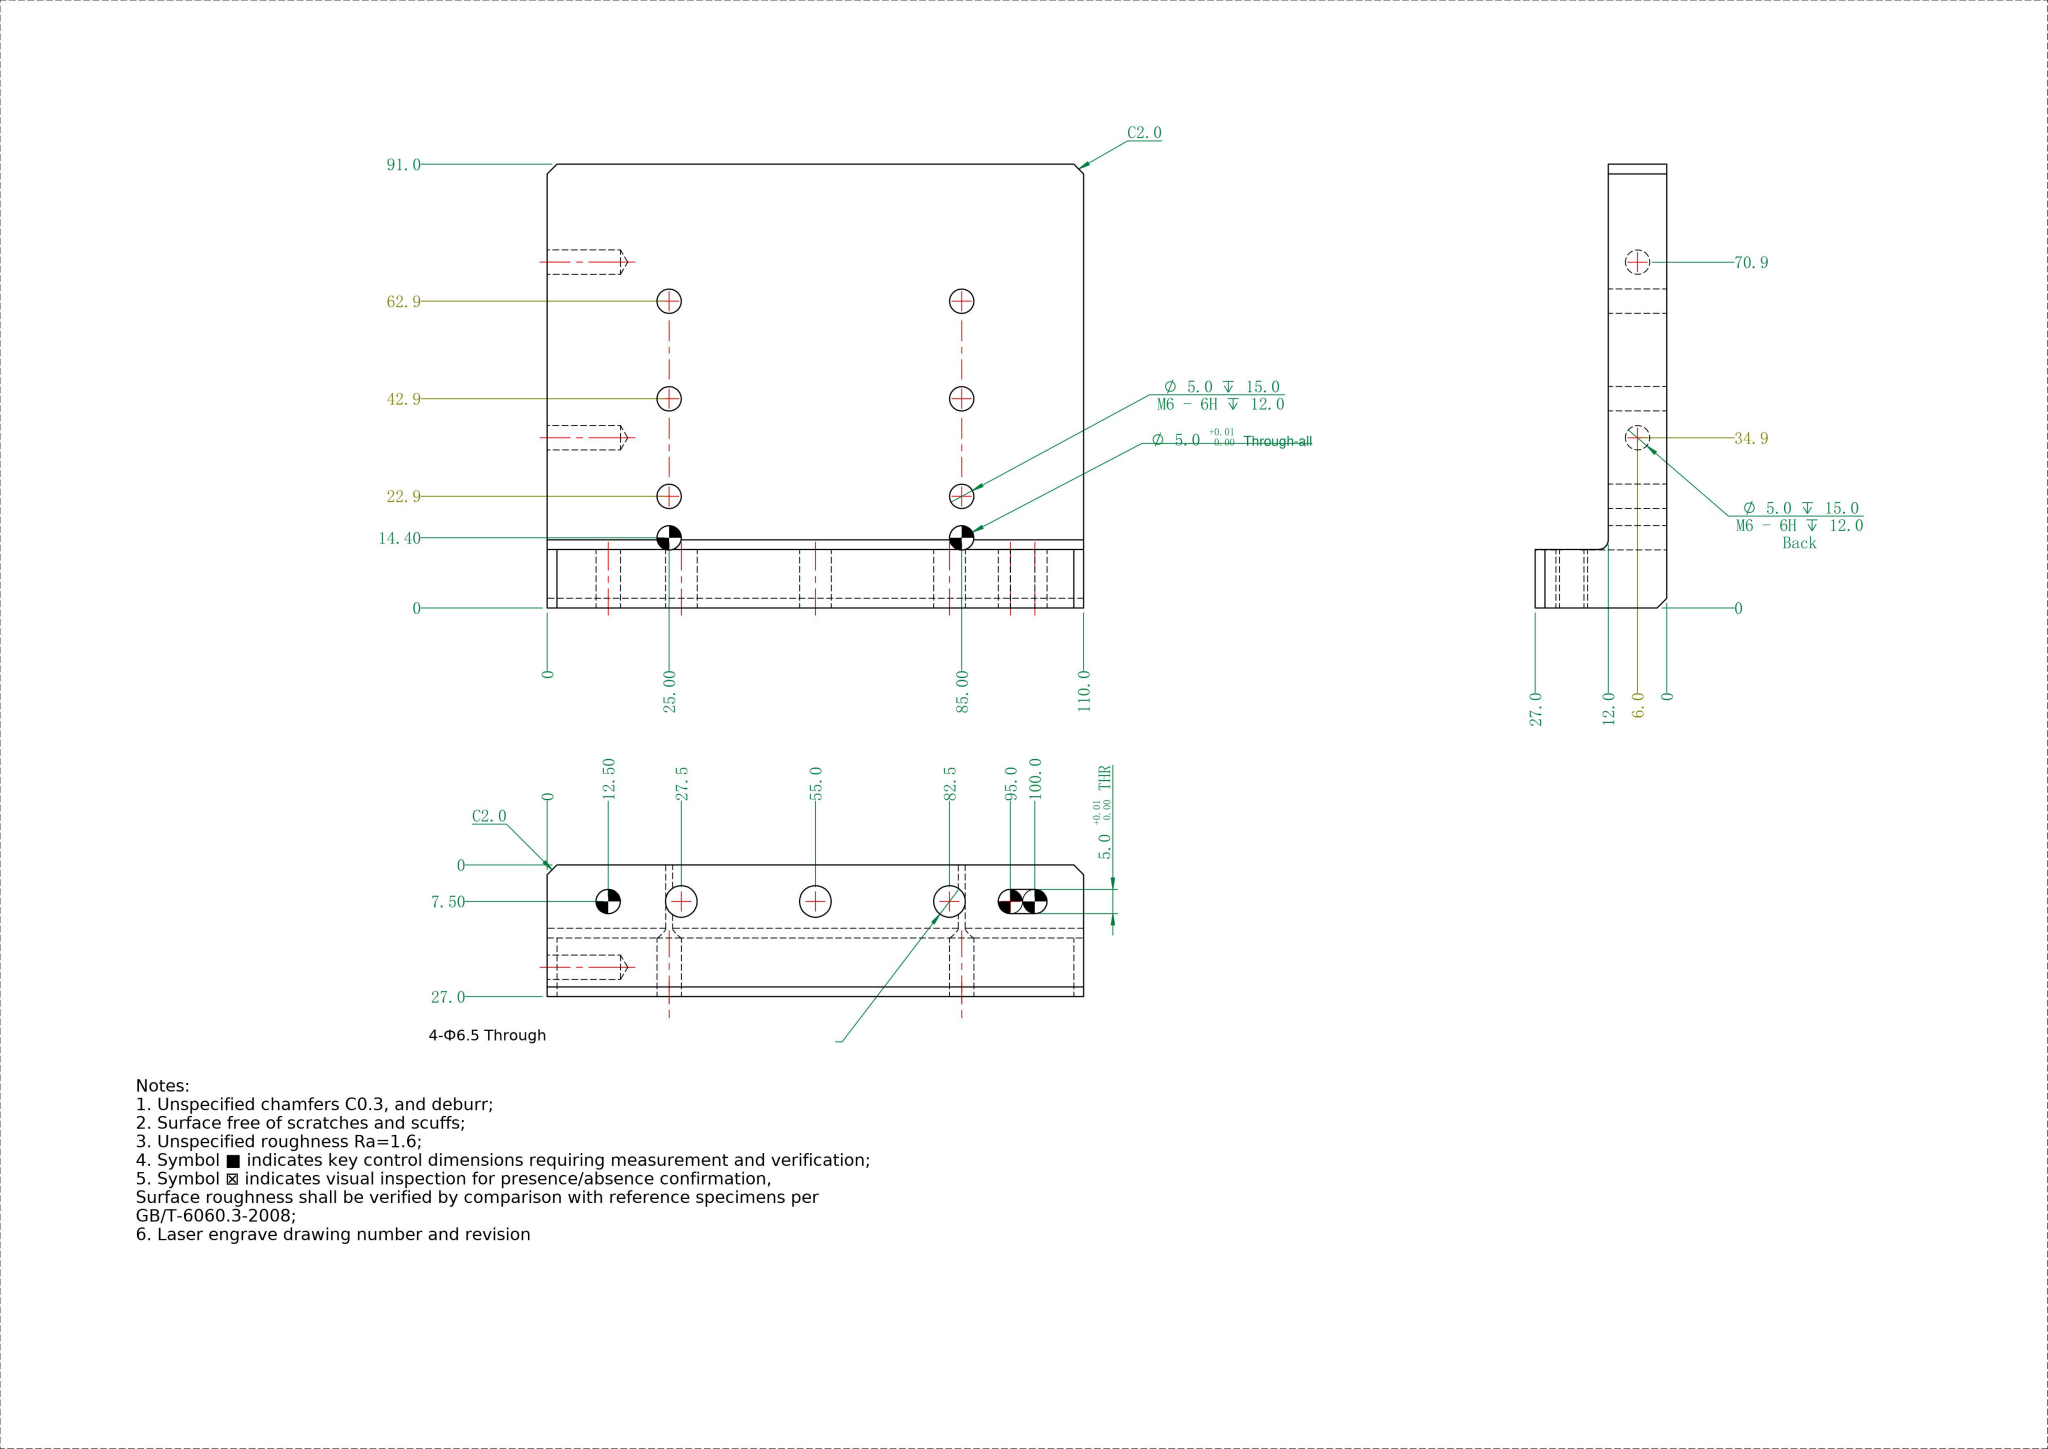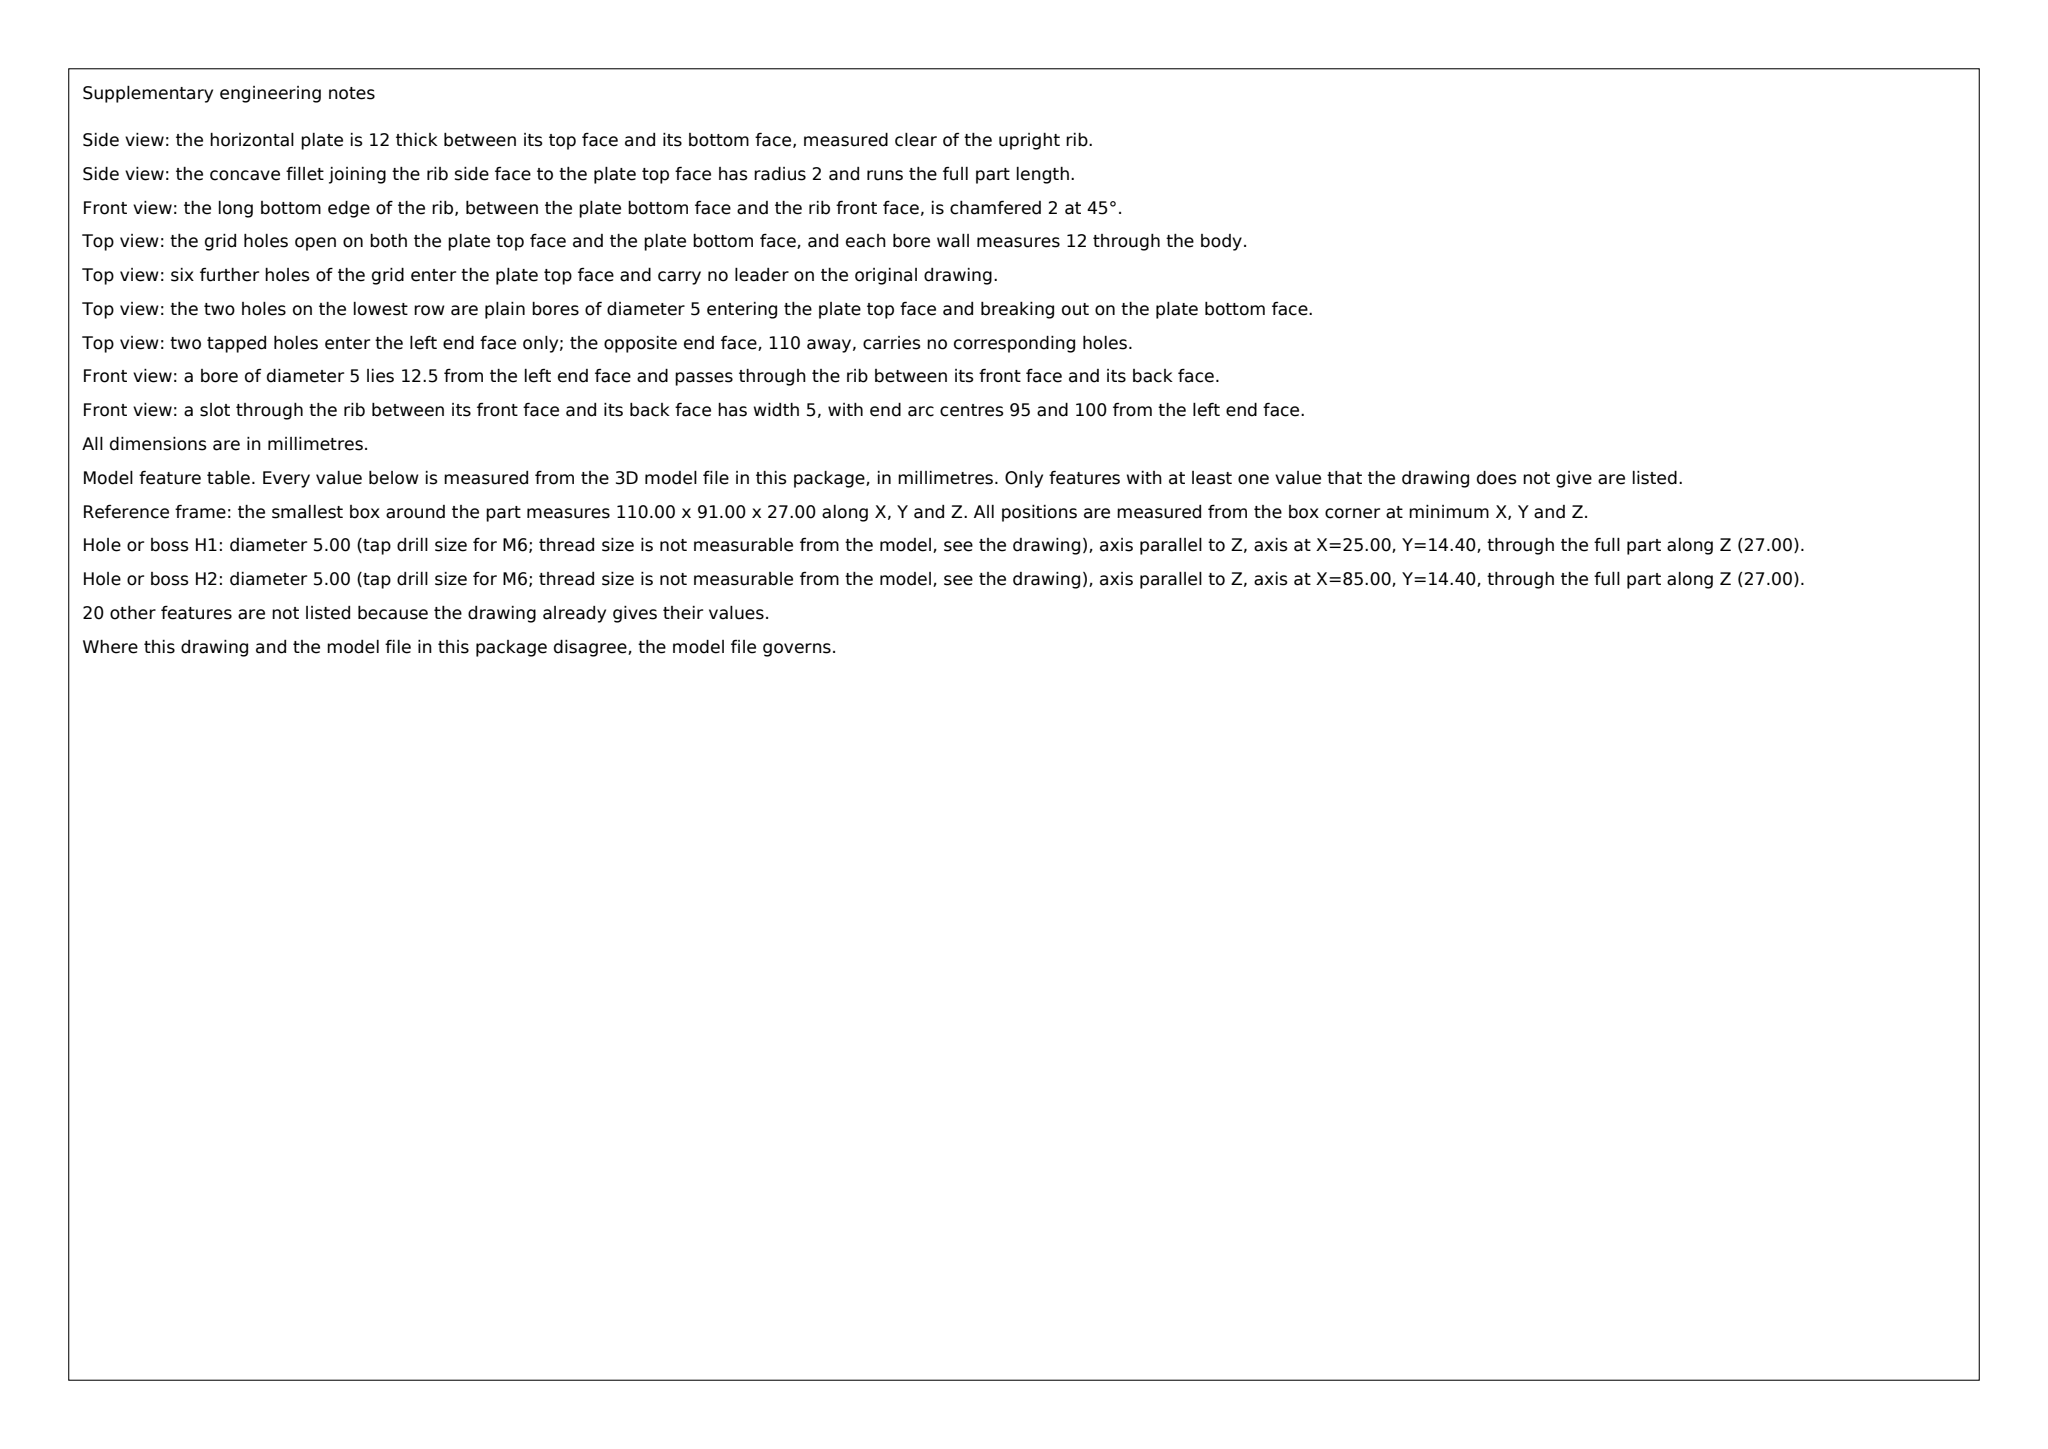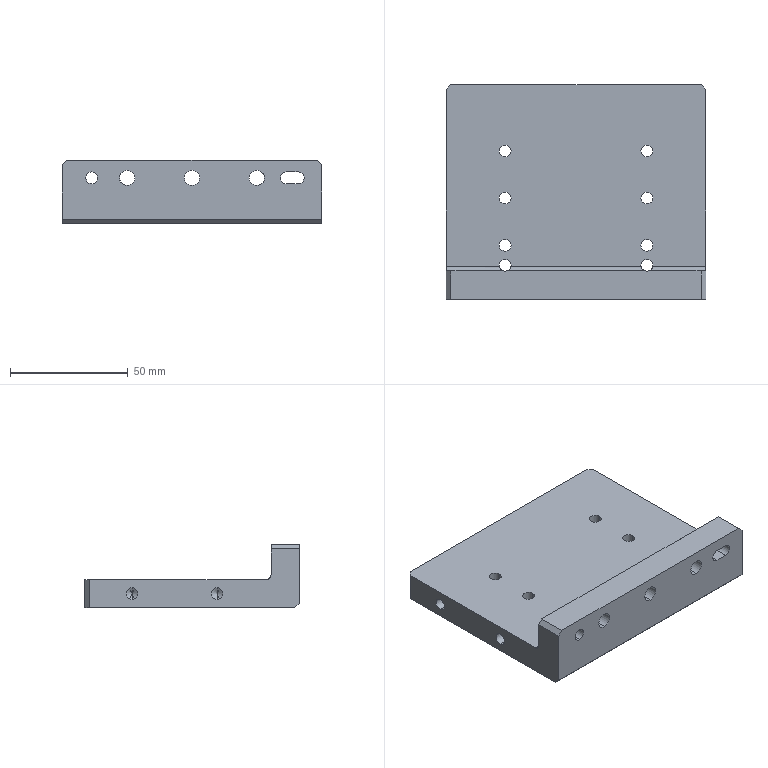Part | SolidWorks | mm | 1 solid | 56 faces | box 110 x 91 x 27 mm | volume 135232 mm3 | cylinder 35 | plane 17 | cone 4 | commonest cylinder face diameters 5 x26 6.5 x6 4 x3
Drawing notes:
3X Ø4.0 cross-hole, axis parallel to X at Y=14.0, Z=14.0 from the bbox min corner; segments X 0.0-24.3, X 25.7-84.3, X 85.7-110.0. | from the solid: cylinders: dia 4.0, axis x, axis_pos [-,14.0,14.0], from/to 0.0-24.3, 25.7-84.3, 85.7-110.0
Slot 5.0 wide THRU in Y (Y 0.0 to 12.0), flanks at Z=17.0 and Z=22.0, end radii centres at X=95.0 and X=100.0, Z=19.5 (7.5 below top face Z=27.0). | from the solid: axis_planes z=17.0 and z=22.0, extent x[95.0,100.0] y[0.0,12.0]; cylinders dia 5.0 axis y at [100.0,-,19.5] and [95.0,-,19.5], from 0.0 to 12.0
3X Ø6.5 THRU (not 4X), axis parallel to Y, Z=19.5, at X=27.5, 55.0 and 82.5; through Y 0.0 to 12.0. | from the solid: cylinders: dia 6.5, axis y, axis_pos [27.5/55.0/82.5, -, 19.5], from 0.0 to 12.0
All dimensions in millimetres (mm); overall size 110.0 x 91.0 x 27.0. | from the solid: bbox_xyz [110.0, 91.0, 27.0] (mm)
1X Ø5.0 THRU, axis parallel to Y, at X=12.5, Z=19.5 from bbox min corner; through Y 0.0 to 12.0 (12.0 deep). | from the solid: cylinders: hole/bore, dia 5.0, axis y, axis_pos [12.5, null, 19.5], from 0.0 to 12.0, arc 360
build123d program:
from build123d import *

# Parameters (mm, degrees)
SKETCH1_W                        = 110
SKETCH1_H                        = 91
BOSS_EXTRUDE1_DEPTH              = 12
SKETCH2_W                        = 110
SKETCH2_H                        = 12
BOSS_EXTRUDE2_DEPTH              = 15
FILLET1_R                        = 2
M6_TAPPED_HOLE1_D                = 5
M6_TAPPED_HOLE1_DEPTH            = 15
M6_TAPPED_HOLE1_TIP              = 1.502
M6_TAPPED_HOLE2_AT_2_COUNT       = 2
M6_TAPPED_HOLE2_AT_2_PITCH       = 60
LPATTERN1_COUNT                  = 3
LPATTERN1_PITCH                  = 20
CHAMFER1_SIZE                    = 2
CHAMFER2_SIZE                    = 2
SIZE_MM_DOWEL_PIN_HOLE_2_D       = 5
SKETCH9_R                        = 3.25
CUT_EXTRUDE1_DEPTH               = 100.975
SIZE_MM_DOWEL_PIN_HOLE_2_2_D     = 5
SIZE_MM_DOWEL_PIN_HOLE_2_2_DEPTH = 15
SIZE_MM_DOWEL_PIN_HOLE_2_2_TIP   = 1.502
CUT_EXTRUDE2_DEPTH               = 100.975


with BuildPart() as part:
    # Sketch1 → Boss-Extrude1 (new body)
    with BuildSketch(Plane.XY):
        Rectangle(SKETCH1_W, SKETCH1_H)
    extrude(amount=BOSS_EXTRUDE1_DEPTH)

    # Sketch2 → Boss-Extrude2 (add)
    with BuildSketch(Plane.XY.offset(12)):
        with Locations((0, -39.5)):
            Rectangle(SKETCH2_W, SKETCH2_H)
    extrude(amount=BOSS_EXTRUDE2_DEPTH)

    # Fillet1
    fillet1_edges = [part.edges().sort_by_distance(p)[0] for p in [
        (0, -33.5, 12),
    ]]
    fillet(fillet1_edges, radius=FILLET1_R)

    # M6 Tapped Hole1
    with Locations(Plane.ZY.offset(55)):
        with Locations((6, -10.6), (6, 25.4)):
            Hole(M6_TAPPED_HOLE1_D / 2, depth=M6_TAPPED_HOLE1_DEPTH)
            with Locations((0, 0, -(M6_TAPPED_HOLE1_DEPTH + M6_TAPPED_HOLE1_TIP / 2))):  # 118° drill point
                Cone(0, M6_TAPPED_HOLE1_D / 2, M6_TAPPED_HOLE1_TIP, mode=Mode.SUBTRACT)

    # Sketch6 → M6 Tapped Hole2 (revolve, cut)
    with BuildSketch(Plane(origin=(30, -22.6, 0), x_dir=(0, 1, 0), z_dir=(1, 0, 0))):
        Polygon((0, 0), (0, 16.502), (2.5, 15), (2.5, 0), align=None)
    m6_tapped_hole2 = revolve(axis=Axis((30, -22.6, -6.35), (0, 0, 1)), mode=Mode.SUBTRACT)

    # M6 Tapped Hole2 at 2: M6 Tapped Hole2 ×2
    with Locations(*[(-i * M6_TAPPED_HOLE2_AT_2_PITCH, 0, 0) for i in range(1, M6_TAPPED_HOLE2_AT_2_COUNT)]):
        add(m6_tapped_hole2, mode=Mode.SUBTRACT)

    # LPattern1: M6 Tapped Hole2 ×3
    with Locations(*[(0, i * LPATTERN1_PITCH, 0) for i in range(1, LPATTERN1_COUNT)]):
        add(m6_tapped_hole2, mode=Mode.SUBTRACT)

    # LPattern1 copy 1 sketch → LPattern1 copy 1 (revolve, cut)
    with BuildSketch(Plane(origin=(-30, -2.6, 0), x_dir=(0, 1, 0), z_dir=(1, 0, 0))):
        Polygon((0, 0), (0, 16.502), (2.5, 15), (2.5, 0), align=None)
    revolve(axis=Axis((-30, -2.6, -6.35), (0, 0, 1)), mode=Mode.SUBTRACT)

    # LPattern1 copy 2 sketch → LPattern1 copy 2 (revolve, cut)
    with BuildSketch(Plane(origin=(-30, 17.4, 0), x_dir=(0, 1, 0), z_dir=(1, 0, 0))):
        Polygon((0, 0), (0, 16.502), (2.5, 15), (2.5, 0), align=None)
    revolve(axis=Axis((-30, 17.4, -6.35), (0, 0, 1)), mode=Mode.SUBTRACT)

    # Chamfer1
    chamfer1_edges = [part.edges().sort_by_distance(p)[0] for p in [
        (-55, -39.5, 27),
        (55, -39.5, 27),
        (-55, 45.5, 6),
        (55, 45.5, 6),
    ]]
    chamfer(chamfer1_edges, length=CHAMFER1_SIZE)

    # Chamfer2
    chamfer2_edges = [part.edges().sort_by_distance(p)[0] for p in [
        (0, -45.5, 0),
    ]]
    chamfer(chamfer2_edges, length=CHAMFER2_SIZE)

    # Size mm Dowel Pin Hole 2 (through all)
    with Locations(Plane(origin=(0, 0, 0), x_dir=(-1, 0, 0), z_dir=(0, 0, -1))):
        with Locations((-30, -31.1), (30, -31.1)):
            Hole(SIZE_MM_DOWEL_PIN_HOLE_2_D / 2)

    # Sketch9 → Cut-Extrude1 (cut, through all)
    with BuildSketch(Plane(origin=(0, -33.5, 0), x_dir=(1, 0, 0), z_dir=(0, 1, 0))):
        with Locations(Location((27.5, -19.5, 0), (0, 0, 270))):
            Circle(SKETCH9_R)
        with Locations(Location((-27.5, -19.5, 0), (0, 0, 270))):
            Circle(SKETCH9_R)
        with Locations(Location((0, -19.5, 0), (0, 0, 270))):
            Circle(SKETCH9_R)
    extrude(amount=-CUT_EXTRUDE1_DEPTH, mode=Mode.SUBTRACT)

    # Size mm Dowel Pin Hole 2_2
    with Locations(Plane(origin=(0, -33.5, 0), x_dir=(1, 0, 0), z_dir=(0, 1, 0))):
        with Locations((-42.5, -19.5), (42.5, -19.5)):
            Hole(SIZE_MM_DOWEL_PIN_HOLE_2_2_D / 2, depth=SIZE_MM_DOWEL_PIN_HOLE_2_2_DEPTH)
            with Locations((0, 0, -(SIZE_MM_DOWEL_PIN_HOLE_2_2_DEPTH + SIZE_MM_DOWEL_PIN_HOLE_2_2_TIP / 2))):  # 118° drill point
                Cone(0, SIZE_MM_DOWEL_PIN_HOLE_2_2_D / 2, SIZE_MM_DOWEL_PIN_HOLE_2_2_TIP, mode=Mode.SUBTRACT)

    # Sketch12 → Cut-Extrude2 (cut, through all)
    with BuildSketch(Plane(origin=(0, -33.5, 0), x_dir=(1, 0, 0), z_dir=(0, 1, 0))):
        with BuildLine():
            Line((40, -17), (45, -17))
            ThreePointArc((45, -17), (47.5, -19.5), (45, -22))
            Line((45, -22), (40, -22))
            ThreePointArc((40, -22), (37.5, -19.5), (40, -17))
        make_face()
    extrude(amount=-CUT_EXTRUDE2_DEPTH, mode=Mode.SUBTRACT)


solid = part.part